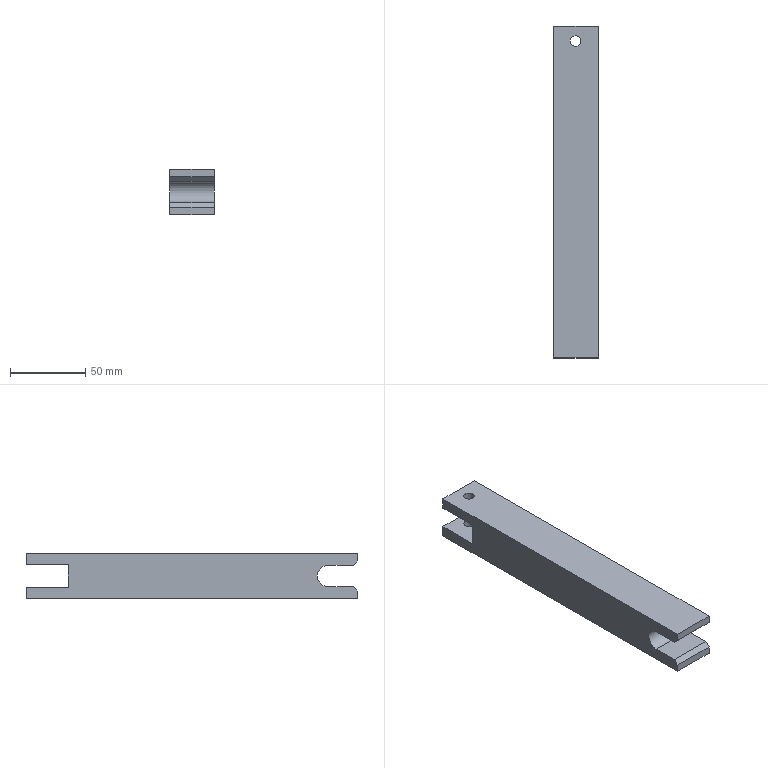Component | NX | CLAMP_PLATE | 1 solid | 18 faces | volume 170937 mm3 | plane 15 | cylinder 3 | commonest cylinder face diameters 7 x2 14 x1